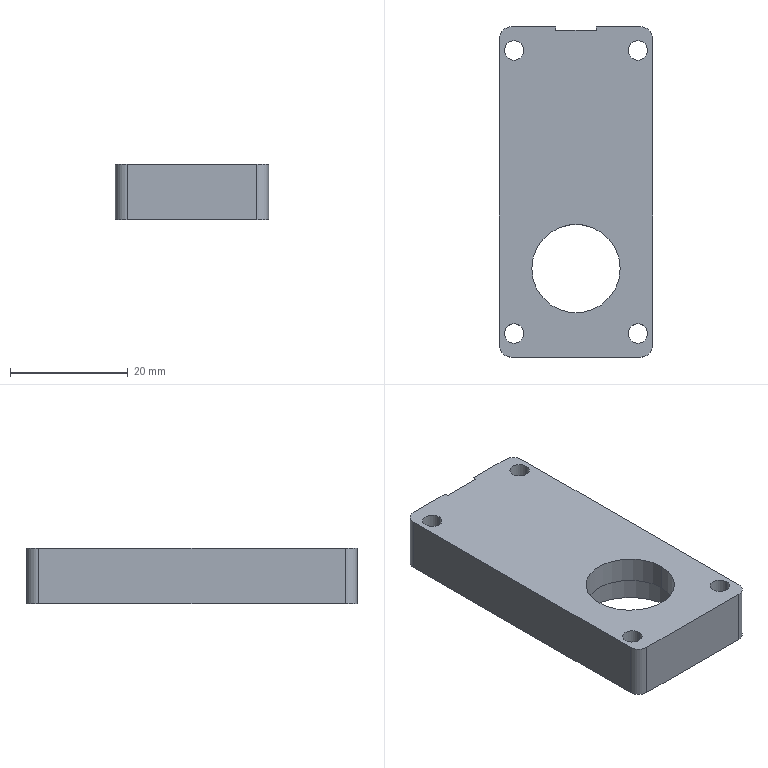Component | SolidWorks | FramePlateSlider.1-1 | 1 solid | 31 faces | box 26 x 56 x 9.4 mm | volume 10956 mm3 | cylinder 20 | plane 9 | cone 2 | commonest cylinder face diameters 3.3 x8 4 x6 19 x2 15 x2 11.6 x2
build123d program:
from build123d import *

# Parameters (mm, degrees)
SKETCH1_2_R           = 7.5
BOSS_EXTRUDE1_DEPTH   = 9.4
M4_TAPPED_HOLE1_D     = 3.3
M4_TAPPED_HOLE1_DEPTH = 10.1
M4_TAPPED_HOLE1_TIP   = 0.9914
M4_TAPPED_HOLE2_D     = 4
M4_TAPPED_HOLE2_DEPTH = 10.1
M4_TAPPED_HOLE2_TIP   = 1.202
SKETCH8_R             = 9.5
CUT_EXTRUDE1_2_DEPTH  = 5
SKETCH1_R             = 5.8
CUT_EXTRUDE1_DEPTH    = 0.6


with BuildPart() as part:
    # Sketch1_2 → Boss-Extrude1 (new body)
    with BuildSketch(Plane.XY):
        with BuildLine():
            Line((-11, 56), (11, 56))
            ThreePointArc((11, 56), (12.414, 55.414), (13, 54))
            Line((13, 54), (13, 2))
            ThreePointArc((13, 2), (12.414, 0.5858), (11, 0))
            Line((11, 0), (-11, 0))
            ThreePointArc((-11, 0), (-12.414, 0.5858), (-13, 2))
            Line((-13, 2), (-13, 54))
            ThreePointArc((-13, 54), (-12.414, 55.414), (-11, 56))
        make_face()
        with Locations((0, 15)):
            Circle(SKETCH1_2_R, mode=Mode.SUBTRACT)
    extrude(amount=BOSS_EXTRUDE1_DEPTH)

    # M4 Tapped Hole1
    with Locations(Plane(origin=(8.389, 4.857, 9.4), x_dir=(1, 0, 0), z_dir=(0, 0, 1))):
        with Locations((-18.889, 47.143), (2.111, 47.143), (-18.889, -0.8568), (2.111, -0.8568)):
            Hole(M4_TAPPED_HOLE1_D / 2, depth=M4_TAPPED_HOLE1_DEPTH)
            with Locations((0, 0, -(M4_TAPPED_HOLE1_DEPTH + M4_TAPPED_HOLE1_TIP / 2))):  # 118° drill point
                Cone(0, M4_TAPPED_HOLE1_D / 2, M4_TAPPED_HOLE1_TIP, mode=Mode.SUBTRACT)

    # M4 Tapped Hole2
    with Locations(Plane(origin=(0, 56, 0), x_dir=(-1, 0, 0), z_dir=(0, 1, 0))):
        with Locations((0, 4.7)):
            Hole(M4_TAPPED_HOLE2_D / 2, depth=M4_TAPPED_HOLE2_DEPTH)
            with Locations((0, 0, -(M4_TAPPED_HOLE2_DEPTH + M4_TAPPED_HOLE2_TIP / 2))):  # 118° drill point
                Cone(0, M4_TAPPED_HOLE2_D / 2, M4_TAPPED_HOLE2_TIP, mode=Mode.SUBTRACT)

    # Sketch8 → Cut-Extrude1_2 (cut)
    with BuildSketch(Plane.XY.offset(9.4)):
        with Locations((0, 15)):
            Circle(SKETCH8_R)
    extrude(amount=-CUT_EXTRUDE1_2_DEPTH, mode=Mode.SUBTRACT)

    # Sketch1 → Cut-Extrude1 (cut, symmetric)
    with BuildSketch(Plane(origin=(0, 56, 0), x_dir=(1, 0, 0), z_dir=(0, 1, 0))):
        with Locations((0, -4.7)):
            Circle(SKETCH1_R)
    extrude(amount=CUT_EXTRUDE1_DEPTH, both=True, mode=Mode.SUBTRACT)


solid = part.part

# Placed as in the assembly
solid = solid.moved(Location((40.5, 151.5, 79.4), (-180, 0, 180)))
STEP:
#1=COLOUR_RGB('',0.7922,0.8196,0.9333);
#2=FILL_AREA_STYLE_COLOUR('',#1);
#3=FILL_AREA_STYLE('',(#2));
#4=SURFACE_STYLE_FILL_AREA(#3);
#5=SURFACE_SIDE_STYLE('',(#4));
#6=SURFACE_STYLE_USAGE(.BOTH.,#5);
#7=PRESENTATION_STYLE_ASSIGNMENT((#6));
#8=CARTESIAN_POINT('',(1.594,7.772,3.02));
#9=VERTEX_POINT('',#8);
#10=CARTESIAN_POINT('',(1.594,7.772,2.862));
#11=VERTEX_POINT('',#10);
#12=CARTESIAN_POINT('',(1.594,7.772,2.941));
#13=DIRECTION('',(-0.,1.,-0.));
#14=DIRECTION('',(0.,0.,-1.));
#15=AXIS2_PLACEMENT_3D('',#12,#13,#14);
#16=CIRCLE('',#15,0.07874);
#17=EDGE_CURVE('',#9,#11,#16,.T.);
#18=ORIENTED_EDGE('',*,*,#17,.F.);
#19=CARTESIAN_POINT('',(1.594,8.146,3.02));
#20=VERTEX_POINT('',#19);
#21=CARTESIAN_POINT('',(1.594,8.169,3.02));
#22=DIRECTION('',(-0.,1.,-0.));
#23=VECTOR('',#22,39.37);
#24=LINE('',#21,#23);
#25=EDGE_CURVE('',#9,#20,#24,.T.);
#26=ORIENTED_EDGE('',*,*,#25,.T.);
#27=CARTESIAN_POINT('',(1.594,8.146,2.862));
#28=VERTEX_POINT('',#27);
#29=CARTESIAN_POINT('',(1.594,8.146,2.941));
#30=DIRECTION('',(0.,-1.,0.));
#31=DIRECTION('',(0.,0.,-1.));
#32=AXIS2_PLACEMENT_3D('',#29,#30,#31);
#33=CIRCLE('',#32,0.07874);
#34=EDGE_CURVE('',#28,#20,#33,.T.);
#35=ORIENTED_EDGE('',*,*,#34,.F.);
#36=CARTESIAN_POINT('',(1.594,8.169,2.862));
#37=DIRECTION('',(-0.,1.,-0.));
#38=VECTOR('',#37,39.37);
#39=LINE('',#36,#38);
#40=EDGE_CURVE('',#11,#28,#39,.T.);
#41=ORIENTED_EDGE('',*,*,#40,.F.);
#42=EDGE_LOOP('',(#18,#26,#35,#41));
#43=FACE_OUTER_BOUND('',#42,.T.);
#44=CARTESIAN_POINT('',(1.594,8.169,2.941));
#45=DIRECTION('',(-0.,1.,-0.));
#46=DIRECTION('',(0.,0.,-1.));
#47=AXIS2_PLACEMENT_3D('',#44,#45,#46);
#48=CYLINDRICAL_SURFACE('',#47,0.07874);
#49=ADVANCED_FACE('',(#43),#48,.F.);
#50=CARTESIAN_POINT('',(1.594,7.724,2.941));
#51=VERTEX_POINT('',#50);
#52=CARTESIAN_POINT('',(1.594,7.772,2.862));
#53=DIRECTION('',(0.,0.515,-0.8572));
#54=VECTOR('',#53,39.37);
#55=LINE('',#52,#54);
#56=EDGE_CURVE('',#51,#11,#55,.T.);
#57=ORIENTED_EDGE('',*,*,#56,.F.);
#58=CARTESIAN_POINT('',(1.594,7.772,3.02));
#59=DIRECTION('',(-0.,0.515,0.8572));
#60=VECTOR('',#59,39.37);
#61=LINE('',#58,#60);
#62=EDGE_CURVE('',#51,#9,#61,.T.);
#63=ORIENTED_EDGE('',*,*,#62,.T.);
#64=ORIENTED_EDGE('',*,*,#17,.T.);
#65=EDGE_LOOP('',(#57,#63,#64));
#66=FACE_OUTER_BOUND('',#65,.T.);
#67=CARTESIAN_POINT('',(1.594,7.772,2.941));
#68=DIRECTION('',(-0.,1.,-0.));
#69=DIRECTION('',(0.,0.,-1.));
#70=AXIS2_PLACEMENT_3D('',#67,#68,#69);
#71=CONICAL_SURFACE('',#70,0.07874,1.03);
#72=ADVANCED_FACE('',(#66),#71,.F.);
#73=CARTESIAN_POINT('',(1.969,6.555,2.953));
#74=VERTEX_POINT('',#73);
#75=CARTESIAN_POINT('',(1.22,6.555,2.953));
#76=VERTEX_POINT('',#75);
#77=CARTESIAN_POINT('',(1.594,6.555,2.953));
#78=DIRECTION('',(0.,-0.,-1.));
#79=DIRECTION('',(-1.,0.,0.));
#80=AXIS2_PLACEMENT_3D('',#77,#78,#79);
#81=CIRCLE('',#80,0.374);
#82=EDGE_CURVE('',#74,#76,#81,.T.);
#83=ORIENTED_EDGE('',*,*,#82,.F.);
#84=CARTESIAN_POINT('',(1.969,6.555,2.756));
#85=VERTEX_POINT('',#84);
#86=CARTESIAN_POINT('',(1.969,6.555,2.953));
#87=DIRECTION('',(0.,-0.,-1.));
#88=VECTOR('',#87,39.37);
#89=LINE('',#86,#88);
#90=EDGE_CURVE('',#74,#85,#89,.T.);
#91=ORIENTED_EDGE('',*,*,#90,.T.);
#92=CARTESIAN_POINT('',(1.22,6.555,2.756));
#93=VERTEX_POINT('',#92);
#94=CARTESIAN_POINT('',(1.594,6.555,2.756));
#95=DIRECTION('',(0.,-0.,-1.));
#96=DIRECTION('',(-1.,0.,0.));
#97=AXIS2_PLACEMENT_3D('',#94,#95,#96);
#98=CIRCLE('',#97,0.374);
#99=EDGE_CURVE('',#85,#93,#98,.T.);
#100=ORIENTED_EDGE('',*,*,#99,.T.);
#101=CARTESIAN_POINT('',(1.22,6.555,2.953));
#102=DIRECTION('',(0.,-0.,-1.));
#103=VECTOR('',#102,39.37);
#104=LINE('',#101,#103);
#105=EDGE_CURVE('',#76,#93,#104,.T.);
#106=ORIENTED_EDGE('',*,*,#105,.F.);
#107=EDGE_LOOP('',(#83,#91,#100,#106));
#108=FACE_OUTER_BOUND('',#107,.T.);
#109=CARTESIAN_POINT('',(1.594,6.555,2.953));
#110=DIRECTION('',(0.,-0.,-1.));
#111=DIRECTION('',(-1.,0.,0.));
#112=AXIS2_PLACEMENT_3D('',#109,#110,#111);
#113=CYLINDRICAL_SURFACE('',#112,0.374);
#114=ADVANCED_FACE('',(#108),#113,.F.);
#115=CARTESIAN_POINT('',(2.073,8.012,3.126));
#116=VERTEX_POINT('',#115);
#117=CARTESIAN_POINT('',(1.943,8.012,3.126));
#118=VERTEX_POINT('',#117);
#119=CARTESIAN_POINT('',(2.008,8.012,3.126));
#120=DIRECTION('',(0.,-0.,-1.));
#121=DIRECTION('',(-1.,0.,0.));
#122=AXIS2_PLACEMENT_3D('',#119,#120,#121);
#123=CIRCLE('',#122,0.06496);
#124=EDGE_CURVE('',#116,#118,#123,.T.);
#125=ORIENTED_EDGE('',*,*,#124,.F.);
#126=CARTESIAN_POINT('',(2.073,8.012,2.756));
#127=VERTEX_POINT('',#126);
#128=CARTESIAN_POINT('',(2.073,8.012,2.756));
#129=DIRECTION('',(0.,-0.,-1.));
#130=VECTOR('',#129,39.37);
#131=LINE('',#128,#130);
#132=EDGE_CURVE('',#116,#127,#131,.T.);
#133=ORIENTED_EDGE('',*,*,#132,.T.);
#134=CARTESIAN_POINT('',(1.943,8.012,2.756));
#135=VERTEX_POINT('',#134);
#136=CARTESIAN_POINT('',(2.008,8.012,2.756));
#137=DIRECTION('',(0.,-0.,-1.));
#138=DIRECTION('',(-1.,0.,0.));
#139=AXIS2_PLACEMENT_3D('',#136,#137,#138);
#140=CIRCLE('',#139,0.06496);
#141=EDGE_CURVE('',#127,#135,#140,.T.);
#142=ORIENTED_EDGE('',*,*,#141,.T.);
#143=CARTESIAN_POINT('',(1.943,8.012,2.756));
#144=DIRECTION('',(0.,-0.,-1.));
#145=VECTOR('',#144,39.37);
#146=LINE('',#143,#145);
#147=EDGE_CURVE('',#118,#135,#146,.T.);
#148=ORIENTED_EDGE('',*,*,#147,.F.);
#149=EDGE_LOOP('',(#125,#133,#142,#148));
#150=FACE_OUTER_BOUND('',#149,.T.);
#151=CARTESIAN_POINT('',(2.008,8.012,2.756));
#152=DIRECTION('',(0.,-0.,-1.));
#153=DIRECTION('',(-1.,0.,0.));
#154=AXIS2_PLACEMENT_3D('',#151,#152,#153);
#155=CYLINDRICAL_SURFACE('',#154,0.06496);
#156=ADVANCED_FACE('',(#150),#155,.F.);
#157=CARTESIAN_POINT('',(1.246,8.012,3.126));
#158=VERTEX_POINT('',#157);
#159=CARTESIAN_POINT('',(1.116,8.012,3.126));
#160=VERTEX_POINT('',#159);
#161=CARTESIAN_POINT('',(1.181,8.012,3.126));
#162=DIRECTION('',(0.,-0.,-1.));
#163=DIRECTION('',(-1.,0.,0.));
#164=AXIS2_PLACEMENT_3D('',#161,#162,#163);
#165=CIRCLE('',#164,0.06496);
#166=EDGE_CURVE('',#158,#160,#165,.T.);
#167=ORIENTED_EDGE('',*,*,#166,.F.);
#168=CARTESIAN_POINT('',(1.246,8.012,2.756));
#169=VERTEX_POINT('',#168);
#170=CARTESIAN_POINT('',(1.246,8.012,2.756));
#171=DIRECTION('',(0.,-0.,-1.));
#172=VECTOR('',#171,39.37);
#173=LINE('',#170,#172);
#174=EDGE_CURVE('',#158,#169,#173,.T.);
#175=ORIENTED_EDGE('',*,*,#174,.T.);
#176=CARTESIAN_POINT('',(1.116,8.012,2.756));
#177=VERTEX_POINT('',#176);
#178=CARTESIAN_POINT('',(1.181,8.012,2.756));
#179=DIRECTION('',(0.,-0.,-1.));
#180=DIRECTION('',(-1.,0.,0.));
#181=AXIS2_PLACEMENT_3D('',#178,#179,#180);
#182=CIRCLE('',#181,0.06496);
#183=EDGE_CURVE('',#169,#177,#182,.T.);
#184=ORIENTED_EDGE('',*,*,#183,.T.);
#185=CARTESIAN_POINT('',(1.116,8.012,2.756));
#186=DIRECTION('',(0.,-0.,-1.));
#187=VECTOR('',#186,39.37);
#188=LINE('',#185,#187);
#189=EDGE_CURVE('',#160,#177,#188,.T.);
#190=ORIENTED_EDGE('',*,*,#189,.F.);
#191=EDGE_LOOP('',(#167,#175,#184,#190));
#192=FACE_OUTER_BOUND('',#191,.T.);
#193=CARTESIAN_POINT('',(1.181,8.012,2.756));
#194=DIRECTION('',(0.,-0.,-1.));
#195=DIRECTION('',(-1.,0.,0.));
#196=AXIS2_PLACEMENT_3D('',#193,#194,#195);
#197=CYLINDRICAL_SURFACE('',#196,0.06496);
#198=ADVANCED_FACE('',(#192),#197,.F.);
#199=CARTESIAN_POINT('',(2.073,6.122,3.126));
#200=VERTEX_POINT('',#199);
#201=CARTESIAN_POINT('',(1.943,6.122,3.126));
#202=VERTEX_POINT('',#201);
#203=CARTESIAN_POINT('',(2.008,6.122,3.126));
#204=DIRECTION('',(0.,-0.,-1.));
#205=DIRECTION('',(-1.,0.,0.));
#206=AXIS2_PLACEMENT_3D('',#203,#204,#205);
#207=CIRCLE('',#206,0.06496);
#208=EDGE_CURVE('',#200,#202,#207,.T.);
#209=ORIENTED_EDGE('',*,*,#208,.F.);
#210=CARTESIAN_POINT('',(2.073,6.122,2.756));
#211=VERTEX_POINT('',#210);
#212=CARTESIAN_POINT('',(2.073,6.122,2.756));
#213=DIRECTION('',(0.,-0.,-1.));
#214=VECTOR('',#213,39.37);
#215=LINE('',#212,#214);
#216=EDGE_CURVE('',#200,#211,#215,.T.);
#217=ORIENTED_EDGE('',*,*,#216,.T.);
#218=CARTESIAN_POINT('',(1.943,6.122,2.756));
#219=VERTEX_POINT('',#218);
#220=CARTESIAN_POINT('',(2.008,6.122,2.756));
#221=DIRECTION('',(0.,-0.,-1.));
#222=DIRECTION('',(-1.,0.,0.));
#223=AXIS2_PLACEMENT_3D('',#220,#221,#222);
#224=CIRCLE('',#223,0.06496);
#225=EDGE_CURVE('',#211,#219,#224,.T.);
#226=ORIENTED_EDGE('',*,*,#225,.T.);
#227=CARTESIAN_POINT('',(1.943,6.122,2.756));
#228=DIRECTION('',(0.,-0.,-1.));
#229=VECTOR('',#228,39.37);
#230=LINE('',#227,#229);
#231=EDGE_CURVE('',#202,#219,#230,.T.);
#232=ORIENTED_EDGE('',*,*,#231,.F.);
#233=EDGE_LOOP('',(#209,#217,#226,#232));
#234=FACE_OUTER_BOUND('',#233,.T.);
#235=CARTESIAN_POINT('',(2.008,6.122,2.756));
#236=DIRECTION('',(0.,-0.,-1.));
#237=DIRECTION('',(-1.,0.,0.));
#238=AXIS2_PLACEMENT_3D('',#235,#236,#237);
#239=CYLINDRICAL_SURFACE('',#238,0.06496);
#240=ADVANCED_FACE('',(#234),#239,.F.);
#241=CARTESIAN_POINT('',(1.246,6.122,3.126));
#242=VERTEX_POINT('',#241);
#243=CARTESIAN_POINT('',(1.116,6.122,3.126));
#244=VERTEX_POINT('',#243);
#245=CARTESIAN_POINT('',(1.181,6.122,3.126));
#246=DIRECTION('',(0.,-0.,-1.));
#247=DIRECTION('',(-1.,0.,0.));
#248=AXIS2_PLACEMENT_3D('',#245,#246,#247);
#249=CIRCLE('',#248,0.06496);
#250=EDGE_CURVE('',#242,#244,#249,.T.);
#251=ORIENTED_EDGE('',*,*,#250,.F.);
#252=CARTESIAN_POINT('',(1.246,6.122,2.756));
#253=VERTEX_POINT('',#252);
#254=CARTESIAN_POINT('',(1.246,6.122,2.756));
#255=DIRECTION('',(0.,-0.,-1.));
#256=VECTOR('',#255,39.37);
#257=LINE('',#254,#256);
#258=EDGE_CURVE('',#242,#253,#257,.T.);
#259=ORIENTED_EDGE('',*,*,#258,.T.);
#260=CARTESIAN_POINT('',(1.116,6.122,2.756));
#261=VERTEX_POINT('',#260);
#262=CARTESIAN_POINT('',(1.181,6.122,2.756));
#263=DIRECTION('',(0.,-0.,-1.));
#264=DIRECTION('',(-1.,0.,0.));
#265=AXIS2_PLACEMENT_3D('',#262,#263,#264);
#266=CIRCLE('',#265,0.06496);
#267=EDGE_CURVE('',#253,#261,#266,.T.);
#268=ORIENTED_EDGE('',*,*,#267,.T.);
#269=CARTESIAN_POINT('',(1.116,6.122,2.756));
#270=DIRECTION('',(0.,-0.,-1.));
#271=VECTOR('',#270,39.37);
#272=LINE('',#269,#271);
#273=EDGE_CURVE('',#244,#261,#272,.T.);
#274=ORIENTED_EDGE('',*,*,#273,.F.);
#275=EDGE_LOOP('',(#251,#259,#268,#274));
#276=FACE_OUTER_BOUND('',#275,.T.);
#277=CARTESIAN_POINT('',(1.181,6.122,2.756));
#278=DIRECTION('',(0.,-0.,-1.));
#279=DIRECTION('',(-1.,0.,0.));
#280=AXIS2_PLACEMENT_3D('',#277,#278,#279);
#281=CYLINDRICAL_SURFACE('',#280,0.06496);
#282=ADVANCED_FACE('',(#276),#281,.F.);
#283=CARTESIAN_POINT('',(1.89,6.555,2.953));
#284=VERTEX_POINT('',#283);
#285=CARTESIAN_POINT('',(1.299,6.555,2.953));
#286=VERTEX_POINT('',#285);
#287=CARTESIAN_POINT('',(1.594,6.555,2.953));
#288=DIRECTION('',(0.,-0.,-1.));
#289=DIRECTION('',(-1.,0.,0.));
#290=AXIS2_PLACEMENT_3D('',#287,#288,#289);
#291=CIRCLE('',#290,0.2953);
#292=EDGE_CURVE('',#284,#286,#291,.T.);
#293=ORIENTED_EDGE('',*,*,#292,.T.);
#294=CARTESIAN_POINT('',(1.299,6.555,3.126));
#295=VERTEX_POINT('',#294);
#296=CARTESIAN_POINT('',(1.299,6.555,2.756));
#297=DIRECTION('',(-0.,0.,1.));
#298=VECTOR('',#297,39.37);
#299=LINE('',#296,#298);
#300=EDGE_CURVE('',#286,#295,#299,.T.);
#301=ORIENTED_EDGE('',*,*,#300,.T.);
#302=CARTESIAN_POINT('',(1.89,6.555,3.126));
#303=VERTEX_POINT('',#302);
#304=CARTESIAN_POINT('',(1.594,6.555,3.126));
#305=DIRECTION('',(0.,-0.,-1.));
#306=DIRECTION('',(-1.,0.,0.));
#307=AXIS2_PLACEMENT_3D('',#304,#305,#306);
#308=CIRCLE('',#307,0.2953);
#309=EDGE_CURVE('',#303,#295,#308,.T.);
#310=ORIENTED_EDGE('',*,*,#309,.F.);
#311=CARTESIAN_POINT('',(1.89,6.555,2.756));
#312=DIRECTION('',(-0.,0.,1.));
#313=VECTOR('',#312,39.37);
#314=LINE('',#311,#313);
#315=EDGE_CURVE('',#284,#303,#314,.T.);
#316=ORIENTED_EDGE('',*,*,#315,.F.);
#317=EDGE_LOOP('',(#293,#301,#310,#316));
#318=FACE_OUTER_BOUND('',#317,.T.);
#319=CARTESIAN_POINT('',(1.594,6.555,2.756));
#320=DIRECTION('',(-0.,0.,1.));
#321=DIRECTION('',(1.,0.,0.));
#322=AXIS2_PLACEMENT_3D('',#319,#320,#321);
#323=CYLINDRICAL_SURFACE('',#322,0.2953);
#324=ADVANCED_FACE('',(#318),#323,.F.);
#325=CARTESIAN_POINT('',(1.161,8.169,3.126));
#326=VERTEX_POINT('',#325);
#327=CARTESIAN_POINT('',(1.461,8.169,3.126));
#328=VERTEX_POINT('',#327);
#329=CARTESIAN_POINT('',(2.028,8.169,3.126));
#330=DIRECTION('',(1.,-0.,0.));
#331=VECTOR('',#330,39.37);
#332=LINE('',#329,#331);
#333=EDGE_CURVE('',#326,#328,#332,.T.);
#334=ORIENTED_EDGE('',*,*,#333,.T.);
#335=CARTESIAN_POINT('',(1.461,8.169,2.756));
#336=VERTEX_POINT('',#335);
#337=CARTESIAN_POINT('',(1.594,8.169,2.941));
#338=DIRECTION('',(0.,-1.,0.));
#339=DIRECTION('',(0.,0.,1.));
#340=AXIS2_PLACEMENT_3D('',#337,#338,#339);
#341=CIRCLE('',#340,0.2283);
#342=EDGE_CURVE('',#328,#336,#341,.T.);
#343=ORIENTED_EDGE('',*,*,#342,.T.);
#344=CARTESIAN_POINT('',(1.161,8.169,2.756));
#345=VERTEX_POINT('',#344);
#346=CARTESIAN_POINT('',(2.028,8.169,2.756));
#347=DIRECTION('',(1.,-0.,0.));
#348=VECTOR('',#347,39.37);
#349=LINE('',#346,#348);
#350=EDGE_CURVE('',#345,#336,#349,.T.);
#351=ORIENTED_EDGE('',*,*,#350,.F.);
#352=CARTESIAN_POINT('',(1.161,8.169,2.756));
#353=DIRECTION('',(-0.,0.,1.));
#354=VECTOR('',#353,39.37);
#355=LINE('',#352,#354);
#356=EDGE_CURVE('',#345,#326,#355,.T.);
#357=ORIENTED_EDGE('',*,*,#356,.T.);
#358=EDGE_LOOP('',(#334,#343,#351,#357));
#359=FACE_OUTER_BOUND('',#358,.T.);
#360=CARTESIAN_POINT('',(2.028,8.169,2.756));
#361=DIRECTION('',(0.,-1.,0.));
#362=DIRECTION('',(-0.,0.,1.));
#363=AXIS2_PLACEMENT_3D('',#360,#361,#362);
#364=PLANE('',#363);
#365=ADVANCED_FACE('',(#359),#364,.F.);
#366=ORIENTED_EDGE('',*,*,#300,.F.);
#367=CARTESIAN_POINT('',(1.594,6.555,2.953));
#368=DIRECTION('',(0.,-0.,-1.));
#369=DIRECTION('',(-1.,0.,0.));
#370=AXIS2_PLACEMENT_3D('',#367,#368,#369);
#371=CIRCLE('',#370,0.2953);
#372=EDGE_CURVE('',#286,#284,#371,.T.);
#373=ORIENTED_EDGE('',*,*,#372,.T.);
#374=ORIENTED_EDGE('',*,*,#315,.T.);
#375=CARTESIAN_POINT('',(1.594,6.555,3.126));
#376=DIRECTION('',(0.,-0.,-1.));
#377=DIRECTION('',(-1.,0.,0.));
#378=AXIS2_PLACEMENT_3D('',#375,#376,#377);
#379=CIRCLE('',#378,0.2953);
#380=EDGE_CURVE('',#295,#303,#379,.T.);
#381=ORIENTED_EDGE('',*,*,#380,.F.);
#382=EDGE_LOOP('',(#366,#373,#374,#381));
#383=FACE_OUTER_BOUND('',#382,.T.);
#384=CARTESIAN_POINT('',(1.594,6.555,2.756));
#385=DIRECTION('',(-0.,0.,1.));
#386=DIRECTION('',(1.,0.,0.));
#387=AXIS2_PLACEMENT_3D('',#384,#385,#386);
#388=CYLINDRICAL_SURFACE('',#387,0.2953);
#389=ADVANCED_FACE('',(#383),#388,.F.);
#390=CARTESIAN_POINT('',(1.461,8.146,2.756));
#391=VERTEX_POINT('',#390);
#392=CARTESIAN_POINT('',(1.461,8.146,2.756));
#393=DIRECTION('',(-0.,1.,-0.));
#394=VECTOR('',#393,39.37);
#395=LINE('',#392,#394);
#396=EDGE_CURVE('',#391,#336,#395,.T.);
#397=ORIENTED_EDGE('',*,*,#396,.F.);
#398=CARTESIAN_POINT('',(1.728,8.146,2.756));
#399=VERTEX_POINT('',#398);
#400=CARTESIAN_POINT('',(1.161,8.146,2.756));
#401=DIRECTION('',(1.,-0.,0.));
#402=VECTOR('',#401,39.37);
#403=LINE('',#400,#402);
#404=EDGE_CURVE('',#391,#399,#403,.T.);
#405=ORIENTED_EDGE('',*,*,#404,.T.);
#406=CARTESIAN_POINT('',(1.728,8.169,2.756));
#407=VERTEX_POINT('',#406);
#408=CARTESIAN_POINT('',(1.728,8.146,2.756));
#409=DIRECTION('',(0.,-1.,0.));
#410=VECTOR('',#409,39.37);
#411=LINE('',#408,#410);
#412=EDGE_CURVE('',#407,#399,#411,.T.);
#413=ORIENTED_EDGE('',*,*,#412,.F.);
#414=CARTESIAN_POINT('',(2.028,8.169,2.756));
#415=VERTEX_POINT('',#414);
#416=CARTESIAN_POINT('',(2.028,8.169,2.756));
#417=DIRECTION('',(1.,-0.,0.));
#418=VECTOR('',#417,39.37);
#419=LINE('',#416,#418);
#420=EDGE_CURVE('',#407,#415,#419,.T.);
#421=ORIENTED_EDGE('',*,*,#420,.T.);
#422=CARTESIAN_POINT('',(2.106,8.091,2.756));
#423=VERTEX_POINT('',#422);
#424=CARTESIAN_POINT('',(2.028,8.091,2.756));
#425=DIRECTION('',(0.,-0.,-1.));
#426=DIRECTION('',(-1.,0.,0.));
#427=AXIS2_PLACEMENT_3D('',#424,#425,#426);
#428=CIRCLE('',#427,0.07874);
#429=EDGE_CURVE('',#415,#423,#428,.T.);
#430=ORIENTED_EDGE('',*,*,#429,.T.);
#431=CARTESIAN_POINT('',(2.106,6.043,2.756));
#432=VERTEX_POINT('',#431);
#433=CARTESIAN_POINT('',(2.106,8.091,2.756));
#434=DIRECTION('',(-0.,-1.,0.));
#435=VECTOR('',#434,39.37);
#436=LINE('',#433,#435);
#437=EDGE_CURVE('',#423,#432,#436,.T.);
#438=ORIENTED_EDGE('',*,*,#437,.T.);
#439=CARTESIAN_POINT('',(2.028,5.965,2.756));
#440=VERTEX_POINT('',#439);
#441=CARTESIAN_POINT('',(2.028,6.043,2.756));
#442=DIRECTION('',(0.,-0.,-1.));
#443=DIRECTION('',(1.,0.,0.));
#444=AXIS2_PLACEMENT_3D('',#441,#442,#443);
#445=CIRCLE('',#444,0.07874);
#446=EDGE_CURVE('',#432,#440,#445,.T.);
#447=ORIENTED_EDGE('',*,*,#446,.T.);
#448=CARTESIAN_POINT('',(1.161,5.965,2.756));
#449=VERTEX_POINT('',#448);
#450=CARTESIAN_POINT('',(2.028,5.965,2.756));
#451=DIRECTION('',(-1.,0.,-0.));
#452=VECTOR('',#451,39.37);
#453=LINE('',#450,#452);
#454=EDGE_CURVE('',#440,#449,#453,.T.);
#455=ORIENTED_EDGE('',*,*,#454,.T.);
#456=CARTESIAN_POINT('',(1.083,6.043,2.756));
#457=VERTEX_POINT('',#456);
#458=CARTESIAN_POINT('',(1.161,6.043,2.756));
#459=DIRECTION('',(0.,-0.,-1.));
#460=DIRECTION('',(-1.,0.,0.));
#461=AXIS2_PLACEMENT_3D('',#458,#459,#460);
#462=CIRCLE('',#461,0.07874);
#463=EDGE_CURVE('',#449,#457,#462,.T.);
#464=ORIENTED_EDGE('',*,*,#463,.T.);
#465=CARTESIAN_POINT('',(1.083,8.091,2.756));
#466=VERTEX_POINT('',#465);
#467=CARTESIAN_POINT('',(1.083,8.091,2.756));
#468=DIRECTION('',(0.,1.,-0.));
#469=VECTOR('',#468,39.37);
#470=LINE('',#467,#469);
#471=EDGE_CURVE('',#457,#466,#470,.T.);
#472=ORIENTED_EDGE('',*,*,#471,.T.);
#473=CARTESIAN_POINT('',(1.161,8.091,2.756));
#474=DIRECTION('',(0.,-0.,-1.));
#475=DIRECTION('',(-1.,0.,0.));
#476=AXIS2_PLACEMENT_3D('',#473,#474,#475);
#477=CIRCLE('',#476,0.07874);
#478=EDGE_CURVE('',#466,#345,#477,.T.);
#479=ORIENTED_EDGE('',*,*,#478,.T.);
#480=ORIENTED_EDGE('',*,*,#350,.T.);
#481=EDGE_LOOP('',(#397,#405,#413,#421,#430,#438,#447,#455,#464,#472,#479,#480));
#482=FACE_OUTER_BOUND('',#481,.T.);
#483=CARTESIAN_POINT('',(1.594,6.555,2.756));
#484=DIRECTION('',(0.,-0.,-1.));
#485=DIRECTION('',(-1.,0.,0.));
#486=AXIS2_PLACEMENT_3D('',#483,#484,#485);
#487=CIRCLE('',#486,0.374);
#488=EDGE_CURVE('',#93,#85,#487,.T.);
#489=ORIENTED_EDGE('',*,*,#488,.F.);
#490=ORIENTED_EDGE('',*,*,#99,.F.);
#491=EDGE_LOOP('',(#489,#490));
#492=FACE_BOUND('',#491,.T.);
#493=CARTESIAN_POINT('',(2.008,8.012,2.756));
#494=DIRECTION('',(0.,-0.,-1.));
#495=DIRECTION('',(-1.,0.,0.));
#496=AXIS2_PLACEMENT_3D('',#493,#494,#495);
#497=CIRCLE('',#496,0.06496);
#498=EDGE_CURVE('',#135,#127,#497,.T.);
#499=ORIENTED_EDGE('',*,*,#498,.F.);
#500=ORIENTED_EDGE('',*,*,#141,.F.);
#501=EDGE_LOOP('',(#499,#500));
#502=FACE_BOUND('',#501,.T.);
#503=CARTESIAN_POINT('',(1.181,8.012,2.756));
#504=DIRECTION('',(0.,-0.,-1.));
#505=DIRECTION('',(-1.,0.,0.));
#506=AXIS2_PLACEMENT_3D('',#503,#504,#505);
#507=CIRCLE('',#506,0.06496);
#508=EDGE_CURVE('',#177,#169,#507,.T.);
#509=ORIENTED_EDGE('',*,*,#508,.F.);
#510=ORIENTED_EDGE('',*,*,#183,.F.);
#511=EDGE_LOOP('',(#509,#510));
#512=FACE_BOUND('',#511,.T.);
#513=CARTESIAN_POINT('',(2.008,6.122,2.756));
#514=DIRECTION('',(0.,-0.,-1.));
#515=DIRECTION('',(-1.,0.,0.));
#516=AXIS2_PLACEMENT_3D('',#513,#514,#515);
#517=CIRCLE('',#516,0.06496);
#518=EDGE_CURVE('',#219,#211,#517,.T.);
#519=ORIENTED_EDGE('',*,*,#518,.F.);
#520=ORIENTED_EDGE('',*,*,#225,.F.);
#521=EDGE_LOOP('',(#519,#520));
#522=FACE_BOUND('',#521,.T.);
#523=CARTESIAN_POINT('',(1.181,6.122,2.756));
#524=DIRECTION('',(0.,-0.,-1.));
#525=DIRECTION('',(-1.,0.,0.));
#526=AXIS2_PLACEMENT_3D('',#523,#524,#525);
#527=CIRCLE('',#526,0.06496);
#528=EDGE_CURVE('',#261,#253,#527,.T.);
#529=ORIENTED_EDGE('',*,*,#528,.F.);
#530=ORIENTED_EDGE('',*,*,#267,.F.);
#531=EDGE_LOOP('',(#529,#530));
#532=FACE_BOUND('',#531,.T.);
#533=CARTESIAN_POINT('',(1.161,6.043,2.756));
#534=DIRECTION('',(0.,-0.,-1.));
#535=DIRECTION('',(-1.,0.,-0.));
#536=AXIS2_PLACEMENT_3D('',#533,#534,#535);
#537=PLANE('',#536);
#538=ADVANCED_FACE('',(#482,#492,#502,#512,#522,#532),#537,.T.);
#539=CARTESIAN_POINT('',(2.008,8.012,3.126));
#540=DIRECTION('',(0.,-0.,-1.));
#541=DIRECTION('',(-1.,0.,0.));
#542=AXIS2_PLACEMENT_3D('',#539,#540,#541);
#543=CIRCLE('',#542,0.06496);
#544=EDGE_CURVE('',#118,#116,#543,.T.);
#545=ORIENTED_EDGE('',*,*,#544,.T.);
#546=ORIENTED_EDGE('',*,*,#124,.T.);
#547=EDGE_LOOP('',(#545,#546));
#548=FACE_BOUND('',#547,.T.);
#549=CARTESIAN_POINT('',(1.181,8.012,3.126));
#550=DIRECTION('',(0.,-0.,-1.));
#551=DIRECTION('',(-1.,0.,0.));
#552=AXIS2_PLACEMENT_3D('',#549,#550,#551);
#553=CIRCLE('',#552,0.06496);
#554=EDGE_CURVE('',#160,#158,#553,.T.);
#555=ORIENTED_EDGE('',*,*,#554,.T.);
#556=ORIENTED_EDGE('',*,*,#166,.T.);
#557=EDGE_LOOP('',(#555,#556));
#558=FACE_BOUND('',#557,.T.);
#559=CARTESIAN_POINT('',(2.008,6.122,3.126));
#560=DIRECTION('',(0.,-0.,-1.));
#561=DIRECTION('',(-1.,0.,0.));
#562=AXIS2_PLACEMENT_3D('',#559,#560,#561);
#563=CIRCLE('',#562,0.06496);
#564=EDGE_CURVE('',#202,#200,#563,.T.);
#565=ORIENTED_EDGE('',*,*,#564,.T.);
#566=ORIENTED_EDGE('',*,*,#208,.T.);
#567=EDGE_LOOP('',(#565,#566));
#568=FACE_BOUND('',#567,.T.);
#569=CARTESIAN_POINT('',(1.181,6.122,3.126));
#570=DIRECTION('',(0.,-0.,-1.));
#571=DIRECTION('',(-1.,0.,0.));
#572=AXIS2_PLACEMENT_3D('',#569,#570,#571);
#573=CIRCLE('',#572,0.06496);
#574=EDGE_CURVE('',#244,#242,#573,.T.);
#575=ORIENTED_EDGE('',*,*,#574,.T.);
#576=ORIENTED_EDGE('',*,*,#250,.T.);
#577=EDGE_LOOP('',(#575,#576));
#578=FACE_BOUND('',#577,.T.);
#579=CARTESIAN_POINT('',(1.461,8.146,3.126));
#580=VERTEX_POINT('',#579);
#581=CARTESIAN_POINT('',(1.728,8.146,3.126));
#582=VERTEX_POINT('',#581);
#583=CARTESIAN_POINT('',(1.161,8.146,3.126));
#584=DIRECTION('',(1.,-0.,0.));
#585=VECTOR('',#584,39.37);
#586=LINE('',#583,#585);
#587=EDGE_CURVE('',#580,#582,#586,.T.);
#588=ORIENTED_EDGE('',*,*,#587,.F.);
#589=CARTESIAN_POINT('',(1.461,8.146,3.126));
#590=DIRECTION('',(-0.,1.,-0.));
#591=VECTOR('',#590,39.37);
#592=LINE('',#589,#591);
#593=EDGE_CURVE('',#580,#328,#592,.T.);
#594=ORIENTED_EDGE('',*,*,#593,.T.);
#595=ORIENTED_EDGE('',*,*,#333,.F.);
#596=CARTESIAN_POINT('',(1.083,8.091,3.126));
#597=VERTEX_POINT('',#596);
#598=CARTESIAN_POINT('',(1.161,8.091,3.126));
#599=DIRECTION('',(0.,-0.,-1.));
#600=DIRECTION('',(-1.,0.,0.));
#601=AXIS2_PLACEMENT_3D('',#598,#599,#600);
#602=CIRCLE('',#601,0.07874);
#603=EDGE_CURVE('',#597,#326,#602,.T.);
#604=ORIENTED_EDGE('',*,*,#603,.F.);
#605=CARTESIAN_POINT('',(1.083,6.043,3.126));
#606=VERTEX_POINT('',#605);
#607=CARTESIAN_POINT('',(1.083,8.091,3.126));
#608=DIRECTION('',(0.,1.,-0.));
#609=VECTOR('',#608,39.37);
#610=LINE('',#607,#609);
#611=EDGE_CURVE('',#606,#597,#610,.T.);
#612=ORIENTED_EDGE('',*,*,#611,.F.);
#613=CARTESIAN_POINT('',(1.161,5.965,3.126));
#614=VERTEX_POINT('',#613);
#615=CARTESIAN_POINT('',(1.161,6.043,3.126));
#616=DIRECTION('',(0.,-0.,-1.));
#617=DIRECTION('',(-1.,0.,0.));
#618=AXIS2_PLACEMENT_3D('',#615,#616,#617);
#619=CIRCLE('',#618,0.07874);
#620=EDGE_CURVE('',#614,#606,#619,.T.);
#621=ORIENTED_EDGE('',*,*,#620,.F.);
#622=CARTESIAN_POINT('',(2.028,5.965,3.126));
#623=VERTEX_POINT('',#622);
#624=CARTESIAN_POINT('',(2.028,5.965,3.126));
#625=DIRECTION('',(-1.,0.,-0.));
#626=VECTOR('',#625,39.37);
#627=LINE('',#624,#626);
#628=EDGE_CURVE('',#623,#614,#627,.T.);
#629=ORIENTED_EDGE('',*,*,#628,.F.);
#630=CARTESIAN_POINT('',(2.106,6.043,3.126));
#631=VERTEX_POINT('',#630);
#632=CARTESIAN_POINT('',(2.028,6.043,3.126));
#633=DIRECTION('',(0.,-0.,-1.));
#634=DIRECTION('',(1.,0.,0.));
#635=AXIS2_PLACEMENT_3D('',#632,#633,#634);
#636=CIRCLE('',#635,0.07874);
#637=EDGE_CURVE('',#631,#623,#636,.T.);
#638=ORIENTED_EDGE('',*,*,#637,.F.);
#639=CARTESIAN_POINT('',(2.106,8.091,3.126));
#640=VERTEX_POINT('',#639);
#641=CARTESIAN_POINT('',(2.106,8.091,3.126));
#642=DIRECTION('',(-0.,-1.,0.));
#643=VECTOR('',#642,39.37);
#644=LINE('',#641,#643);
#645=EDGE_CURVE('',#640,#631,#644,.T.);
#646=ORIENTED_EDGE('',*,*,#645,.F.);
#647=CARTESIAN_POINT('',(2.028,8.169,3.126));
#648=VERTEX_POINT('',#647);
#649=CARTESIAN_POINT('',(2.028,8.091,3.126));
#650=DIRECTION('',(0.,-0.,-1.));
#651=DIRECTION('',(-1.,0.,0.));
#652=AXIS2_PLACEMENT_3D('',#649,#650,#651);
#653=CIRCLE('',#652,0.07874);
#654=EDGE_CURVE('',#648,#640,#653,.T.);
#655=ORIENTED_EDGE('',*,*,#654,.F.);
#656=CARTESIAN_POINT('',(1.728,8.169,3.126));
#657=VERTEX_POINT('',#656);
#658=CARTESIAN_POINT('',(2.028,8.169,3.126));
#659=DIRECTION('',(1.,-0.,0.));
#660=VECTOR('',#659,39.37);
#661=LINE('',#658,#660);
#662=EDGE_CURVE('',#657,#648,#661,.T.);
#663=ORIENTED_EDGE('',*,*,#662,.F.);
#664=CARTESIAN_POINT('',(1.728,8.146,3.126));
#665=DIRECTION('',(0.,-1.,0.));
#666=VECTOR('',#665,39.37);
#667=LINE('',#664,#666);
#668=EDGE_CURVE('',#657,#582,#667,.T.);
#669=ORIENTED_EDGE('',*,*,#668,.T.);
#670=EDGE_LOOP('',(#588,#594,#595,#604,#612,#621,#629,#638,#646,#655,#663,#669));
#671=FACE_OUTER_BOUND('',#670,.T.);
#672=ORIENTED_EDGE('',*,*,#309,.T.);
#673=ORIENTED_EDGE('',*,*,#380,.T.);
#674=EDGE_LOOP('',(#672,#673));
#675=FACE_BOUND('',#674,.T.);
#676=CARTESIAN_POINT('',(1.161,6.043,3.126));
#677=DIRECTION('',(0.,-0.,-1.));
#678=DIRECTION('',(-1.,0.,-0.));
#679=AXIS2_PLACEMENT_3D('',#676,#677,#678);
#680=PLANE('',#679);
#681=ADVANCED_FACE('',(#548,#558,#568,#578,#671,#675),#680,.F.);
#682=ORIENTED_EDGE('',*,*,#620,.T.);
#683=CARTESIAN_POINT('',(1.083,6.043,2.756));
#684=DIRECTION('',(-0.,0.,1.));
#685=VECTOR('',#684,39.37);
#686=LINE('',#683,#685);
#687=EDGE_CURVE('',#457,#606,#686,.T.);
#688=ORIENTED_EDGE('',*,*,#687,.F.);
#689=ORIENTED_EDGE('',*,*,#463,.F.);
#690=CARTESIAN_POINT('',(1.161,5.965,2.756));
#691=DIRECTION('',(-0.,0.,1.));
#692=VECTOR('',#691,39.37);
#693=LINE('',#690,#692);
#694=EDGE_CURVE('',#449,#614,#693,.T.);
#695=ORIENTED_EDGE('',*,*,#694,.T.);
#696=EDGE_LOOP('',(#682,#688,#689,#695));
#697=FACE_OUTER_BOUND('',#696,.T.);
#698=CARTESIAN_POINT('',(1.161,6.043,2.756));
#699=DIRECTION('',(-0.,0.,1.));
#700=DIRECTION('',(1.,0.,0.));
#701=AXIS2_PLACEMENT_3D('',#698,#699,#700);
#702=CYLINDRICAL_SURFACE('',#701,0.07874);
#703=ADVANCED_FACE('',(#697),#702,.T.);
#704=ORIENTED_EDGE('',*,*,#611,.T.);
#705=CARTESIAN_POINT('',(1.083,8.091,2.756));
#706=DIRECTION('',(-0.,0.,1.));
#707=VECTOR('',#706,39.37);
#708=LINE('',#705,#707);
#709=EDGE_CURVE('',#466,#597,#708,.T.);
#710=ORIENTED_EDGE('',*,*,#709,.F.);
#711=ORIENTED_EDGE('',*,*,#471,.F.);
#712=ORIENTED_EDGE('',*,*,#687,.T.);
#713=EDGE_LOOP('',(#704,#710,#711,#712));
#714=FACE_OUTER_BOUND('',#713,.T.);
#715=CARTESIAN_POINT('',(1.083,8.091,2.756));
#716=DIRECTION('',(1.,-0.,0.));
#717=DIRECTION('',(-0.,-1.,0.));
#718=AXIS2_PLACEMENT_3D('',#715,#716,#717);
#719=PLANE('',#718);
#720=ADVANCED_FACE('',(#714),#719,.F.);
#721=ORIENTED_EDGE('',*,*,#603,.T.);
#722=ORIENTED_EDGE('',*,*,#356,.F.);
#723=ORIENTED_EDGE('',*,*,#478,.F.);
#724=ORIENTED_EDGE('',*,*,#709,.T.);
#725=EDGE_LOOP('',(#721,#722,#723,#724));
#726=FACE_OUTER_BOUND('',#725,.T.);
#727=CARTESIAN_POINT('',(1.161,8.091,2.756));
#728=DIRECTION('',(-0.,0.,1.));
#729=DIRECTION('',(1.,0.,0.));
#730=AXIS2_PLACEMENT_3D('',#727,#728,#729);
#731=CYLINDRICAL_SURFACE('',#730,0.07874);
#732=ADVANCED_FACE('',(#726),#731,.T.);
#733=ORIENTED_EDGE('',*,*,#420,.F.);
#734=CARTESIAN_POINT('',(1.594,8.169,2.941));
#735=DIRECTION('',(0.,-1.,0.));
#736=DIRECTION('',(0.,0.,1.));
#737=AXIS2_PLACEMENT_3D('',#734,#735,#736);
#738=CIRCLE('',#737,0.2283);
#739=EDGE_CURVE('',#407,#657,#738,.T.);
#740=ORIENTED_EDGE('',*,*,#739,.T.);
#741=ORIENTED_EDGE('',*,*,#662,.T.);
#742=CARTESIAN_POINT('',(2.028,8.169,2.756));
#743=DIRECTION('',(-0.,0.,1.));
#744=VECTOR('',#743,39.37);
#745=LINE('',#742,#744);
#746=EDGE_CURVE('',#415,#648,#745,.T.);
#747=ORIENTED_EDGE('',*,*,#746,.F.);
#748=EDGE_LOOP('',(#733,#740,#741,#747));
#749=FACE_OUTER_BOUND('',#748,.T.);
#750=CARTESIAN_POINT('',(2.028,8.169,2.756));
#751=DIRECTION('',(0.,-1.,0.));
#752=DIRECTION('',(-0.,0.,1.));
#753=AXIS2_PLACEMENT_3D('',#750,#751,#752);
#754=PLANE('',#753);
#755=ADVANCED_FACE('',(#749),#754,.F.);
#756=ORIENTED_EDGE('',*,*,#654,.T.);
#757=CARTESIAN_POINT('',(2.106,8.091,2.756));
#758=DIRECTION('',(-0.,0.,1.));
#759=VECTOR('',#758,39.37);
#760=LINE('',#757,#759);
#761=EDGE_CURVE('',#423,#640,#760,.T.);
#762=ORIENTED_EDGE('',*,*,#761,.F.);
#763=ORIENTED_EDGE('',*,*,#429,.F.);
#764=ORIENTED_EDGE('',*,*,#746,.T.);
#765=EDGE_LOOP('',(#756,#762,#763,#764));
#766=FACE_OUTER_BOUND('',#765,.T.);
#767=CARTESIAN_POINT('',(2.028,8.091,2.756));
#768=DIRECTION('',(-0.,0.,1.));
#769=DIRECTION('',(1.,0.,0.));
#770=AXIS2_PLACEMENT_3D('',#767,#768,#769);
#771=CYLINDRICAL_SURFACE('',#770,0.07874);
#772=ADVANCED_FACE('',(#766),#771,.T.);
#773=ORIENTED_EDGE('',*,*,#645,.T.);
#774=CARTESIAN_POINT('',(2.106,6.043,2.756));
#775=DIRECTION('',(-0.,0.,1.));
#776=VECTOR('',#775,39.37);
#777=LINE('',#774,#776);
#778=EDGE_CURVE('',#432,#631,#777,.T.);
#779=ORIENTED_EDGE('',*,*,#778,.F.);
#780=ORIENTED_EDGE('',*,*,#437,.F.);
#781=ORIENTED_EDGE('',*,*,#761,.T.);
#782=EDGE_LOOP('',(#773,#779,#780,#781));
#783=FACE_OUTER_BOUND('',#782,.T.);
#784=CARTESIAN_POINT('',(2.106,8.091,2.756));
#785=DIRECTION('',(-1.,0.,-0.));
#786=DIRECTION('',(0.,1.,-0.));
#787=AXIS2_PLACEMENT_3D('',#784,#785,#786);
#788=PLANE('',#787);
#789=ADVANCED_FACE('',(#783),#788,.F.);
#790=ORIENTED_EDGE('',*,*,#637,.T.);
#791=CARTESIAN_POINT('',(2.028,5.965,2.756));
#792=DIRECTION('',(-0.,0.,1.));
#793=VECTOR('',#792,39.37);
#794=LINE('',#791,#793);
#795=EDGE_CURVE('',#440,#623,#794,.T.);
#796=ORIENTED_EDGE('',*,*,#795,.F.);
#797=ORIENTED_EDGE('',*,*,#446,.F.);
#798=ORIENTED_EDGE('',*,*,#778,.T.);
#799=EDGE_LOOP('',(#790,#796,#797,#798));
#800=FACE_OUTER_BOUND('',#799,.T.);
#801=CARTESIAN_POINT('',(2.028,6.043,2.756));
#802=DIRECTION('',(-0.,0.,1.));
#803=DIRECTION('',(1.,0.,0.));
#804=AXIS2_PLACEMENT_3D('',#801,#802,#803);
#805=CYLINDRICAL_SURFACE('',#804,0.07874);
#806=ADVANCED_FACE('',(#800),#805,.T.);
#807=ORIENTED_EDGE('',*,*,#628,.T.);
#808=ORIENTED_EDGE('',*,*,#694,.F.);
#809=ORIENTED_EDGE('',*,*,#454,.F.);
#810=ORIENTED_EDGE('',*,*,#795,.T.);
#811=EDGE_LOOP('',(#807,#808,#809,#810));
#812=FACE_OUTER_BOUND('',#811,.T.);
#813=CARTESIAN_POINT('',(2.028,5.965,2.756));
#814=DIRECTION('',(-0.,1.,-0.));
#815=DIRECTION('',(0.,-0.,-1.));
#816=AXIS2_PLACEMENT_3D('',#813,#814,#815);
#817=PLANE('',#816);
#818=ADVANCED_FACE('',(#812),#817,.F.);
#819=ORIENTED_EDGE('',*,*,#258,.F.);
#820=ORIENTED_EDGE('',*,*,#574,.F.);
#821=ORIENTED_EDGE('',*,*,#273,.T.);
#822=ORIENTED_EDGE('',*,*,#528,.T.);
#823=EDGE_LOOP('',(#819,#820,#821,#822));
#824=FACE_OUTER_BOUND('',#823,.T.);
#825=CARTESIAN_POINT('',(1.181,6.122,2.756));
#826=DIRECTION('',(0.,-0.,-1.));
#827=DIRECTION('',(-1.,0.,0.));
#828=AXIS2_PLACEMENT_3D('',#825,#826,#827);
#829=CYLINDRICAL_SURFACE('',#828,0.06496);
#830=ADVANCED_FACE('',(#824),#829,.F.);
#831=ORIENTED_EDGE('',*,*,#216,.F.);
#832=ORIENTED_EDGE('',*,*,#564,.F.);
#833=ORIENTED_EDGE('',*,*,#231,.T.);
#834=ORIENTED_EDGE('',*,*,#518,.T.);
#835=EDGE_LOOP('',(#831,#832,#833,#834));
#836=FACE_OUTER_BOUND('',#835,.T.);
#837=CARTESIAN_POINT('',(2.008,6.122,2.756));
#838=DIRECTION('',(0.,-0.,-1.));
#839=DIRECTION('',(-1.,0.,0.));
#840=AXIS2_PLACEMENT_3D('',#837,#838,#839);
#841=CYLINDRICAL_SURFACE('',#840,0.06496);
#842=ADVANCED_FACE('',(#836),#841,.F.);
#843=ORIENTED_EDGE('',*,*,#174,.F.);
#844=ORIENTED_EDGE('',*,*,#554,.F.);
#845=ORIENTED_EDGE('',*,*,#189,.T.);
#846=ORIENTED_EDGE('',*,*,#508,.T.);
#847=EDGE_LOOP('',(#843,#844,#845,#846));
#848=FACE_OUTER_BOUND('',#847,.T.);
#849=CARTESIAN_POINT('',(1.181,8.012,2.756));
#850=DIRECTION('',(0.,-0.,-1.));
#851=DIRECTION('',(-1.,0.,0.));
#852=AXIS2_PLACEMENT_3D('',#849,#850,#851);
#853=CYLINDRICAL_SURFACE('',#852,0.06496);
#854=ADVANCED_FACE('',(#848),#853,.F.);
#855=ORIENTED_EDGE('',*,*,#132,.F.);
#856=ORIENTED_EDGE('',*,*,#544,.F.);
#857=ORIENTED_EDGE('',*,*,#147,.T.);
#858=ORIENTED_EDGE('',*,*,#498,.T.);
#859=EDGE_LOOP('',(#855,#856,#857,#858));
#860=FACE_OUTER_BOUND('',#859,.T.);
#861=CARTESIAN_POINT('',(2.008,8.012,2.756));
#862=DIRECTION('',(0.,-0.,-1.));
#863=DIRECTION('',(-1.,0.,0.));
#864=AXIS2_PLACEMENT_3D('',#861,#862,#863);
#865=CYLINDRICAL_SURFACE('',#864,0.06496);
#866=ADVANCED_FACE('',(#860),#865,.F.);
#867=ORIENTED_EDGE('',*,*,#90,.F.);
#868=CARTESIAN_POINT('',(1.594,6.555,2.953));
#869=DIRECTION('',(0.,-0.,-1.));
#870=DIRECTION('',(-1.,0.,0.));
#871=AXIS2_PLACEMENT_3D('',#868,#869,#870);
#872=CIRCLE('',#871,0.374);
#873=EDGE_CURVE('',#76,#74,#872,.T.);
#874=ORIENTED_EDGE('',*,*,#873,.F.);
#875=ORIENTED_EDGE('',*,*,#105,.T.);
#876=ORIENTED_EDGE('',*,*,#488,.T.);
#877=EDGE_LOOP('',(#867,#874,#875,#876));
#878=FACE_OUTER_BOUND('',#877,.T.);
#879=CARTESIAN_POINT('',(1.594,6.555,2.953));
#880=DIRECTION('',(0.,-0.,-1.));
#881=DIRECTION('',(-1.,0.,0.));
#882=AXIS2_PLACEMENT_3D('',#879,#880,#881);
#883=CYLINDRICAL_SURFACE('',#882,0.374);
#884=ADVANCED_FACE('',(#878),#883,.F.);
#885=ORIENTED_EDGE('',*,*,#292,.F.);
#886=ORIENTED_EDGE('',*,*,#372,.F.);
#887=EDGE_LOOP('',(#885,#886));
#888=FACE_BOUND('',#887,.T.);
#889=ORIENTED_EDGE('',*,*,#873,.T.);
#890=ORIENTED_EDGE('',*,*,#82,.T.);
#891=EDGE_LOOP('',(#889,#890));
#892=FACE_OUTER_BOUND('',#891,.T.);
#893=CARTESIAN_POINT('',(1.594,6.555,2.953));
#894=DIRECTION('',(0.,-0.,-1.));
#895=DIRECTION('',(-1.,0.,-0.));
#896=AXIS2_PLACEMENT_3D('',#893,#894,#895);
#897=PLANE('',#896);
#898=ADVANCED_FACE('',(#888,#892),#897,.T.);
#899=ORIENTED_EDGE('',*,*,#396,.T.);
#900=ORIENTED_EDGE('',*,*,#342,.F.);
#901=ORIENTED_EDGE('',*,*,#593,.F.);
#902=CARTESIAN_POINT('',(1.594,8.146,2.941));
#903=DIRECTION('',(-0.,1.,-0.));
#904=DIRECTION('',(0.,0.,-1.));
#905=AXIS2_PLACEMENT_3D('',#902,#903,#904);
#906=CIRCLE('',#905,0.2283);
#907=EDGE_CURVE('',#391,#580,#906,.T.);
#908=ORIENTED_EDGE('',*,*,#907,.F.);
#909=EDGE_LOOP('',(#899,#900,#901,#908));
#910=FACE_OUTER_BOUND('',#909,.T.);
#911=CARTESIAN_POINT('',(1.594,8.146,2.941));
#912=DIRECTION('',(-0.,1.,-0.));
#913=DIRECTION('',(0.,0.,-1.));
#914=AXIS2_PLACEMENT_3D('',#911,#912,#913);
#915=CYLINDRICAL_SURFACE('',#914,0.2283);
#916=ADVANCED_FACE('',(#910),#915,.F.);
#917=ORIENTED_EDGE('',*,*,#34,.T.);
#918=CARTESIAN_POINT('',(1.594,8.146,2.941));
#919=DIRECTION('',(0.,-1.,0.));
#920=DIRECTION('',(0.,0.,-1.));
#921=AXIS2_PLACEMENT_3D('',#918,#919,#920);
#922=CIRCLE('',#921,0.07874);
#923=EDGE_CURVE('',#20,#28,#922,.T.);
#924=ORIENTED_EDGE('',*,*,#923,.T.);
#925=EDGE_LOOP('',(#917,#924));
#926=FACE_BOUND('',#925,.T.);
#927=ORIENTED_EDGE('',*,*,#907,.T.);
#928=ORIENTED_EDGE('',*,*,#587,.T.);
#929=CARTESIAN_POINT('',(1.594,8.146,2.941));
#930=DIRECTION('',(-0.,1.,-0.));
#931=DIRECTION('',(0.,0.,-1.));
#932=AXIS2_PLACEMENT_3D('',#929,#930,#931);
#933=CIRCLE('',#932,0.2283);
#934=EDGE_CURVE('',#582,#399,#933,.T.);
#935=ORIENTED_EDGE('',*,*,#934,.T.);
#936=ORIENTED_EDGE('',*,*,#404,.F.);
#937=EDGE_LOOP('',(#927,#928,#935,#936));
#938=FACE_OUTER_BOUND('',#937,.T.);
#939=CARTESIAN_POINT('',(1.594,8.146,2.941));
#940=DIRECTION('',(-0.,1.,-0.));
#941=DIRECTION('',(0.,-0.,-1.));
#942=AXIS2_PLACEMENT_3D('',#939,#940,#941);
#943=PLANE('',#942);
#944=ADVANCED_FACE('',(#926,#938),#943,.T.);
#945=ORIENTED_EDGE('',*,*,#412,.T.);
#946=ORIENTED_EDGE('',*,*,#934,.F.);
#947=ORIENTED_EDGE('',*,*,#668,.F.);
#948=ORIENTED_EDGE('',*,*,#739,.F.);
#949=EDGE_LOOP('',(#945,#946,#947,#948));
#950=FACE_OUTER_BOUND('',#949,.T.);
#951=CARTESIAN_POINT('',(1.594,8.146,2.941));
#952=DIRECTION('',(-0.,1.,-0.));
#953=DIRECTION('',(0.,0.,-1.));
#954=AXIS2_PLACEMENT_3D('',#951,#952,#953);
#955=CYLINDRICAL_SURFACE('',#954,0.2283);
#956=ADVANCED_FACE('',(#950),#955,.F.);
#957=ORIENTED_EDGE('',*,*,#62,.F.);
#958=ORIENTED_EDGE('',*,*,#56,.T.);
#959=CARTESIAN_POINT('',(1.594,7.772,2.941));
#960=DIRECTION('',(-0.,1.,-0.));
#961=DIRECTION('',(0.,0.,-1.));
#962=AXIS2_PLACEMENT_3D('',#959,#960,#961);
#963=CIRCLE('',#962,0.07874);
#964=EDGE_CURVE('',#11,#9,#963,.T.);
#965=ORIENTED_EDGE('',*,*,#964,.T.);
#966=EDGE_LOOP('',(#957,#958,#965));
#967=FACE_OUTER_BOUND('',#966,.T.);
#968=CARTESIAN_POINT('',(1.594,7.772,2.941));
#969=DIRECTION('',(-0.,1.,-0.));
#970=DIRECTION('',(0.,0.,-1.));
#971=AXIS2_PLACEMENT_3D('',#968,#969,#970);
#972=CONICAL_SURFACE('',#971,0.07874,1.03);
#973=ADVANCED_FACE('',(#967),#972,.F.);
#974=ORIENTED_EDGE('',*,*,#25,.F.);
#975=ORIENTED_EDGE('',*,*,#964,.F.);
#976=ORIENTED_EDGE('',*,*,#40,.T.);
#977=ORIENTED_EDGE('',*,*,#923,.F.);
#978=EDGE_LOOP('',(#974,#975,#976,#977));
#979=FACE_OUTER_BOUND('',#978,.T.);
#980=CARTESIAN_POINT('',(1.594,8.169,2.941));
#981=DIRECTION('',(-0.,1.,-0.));
#982=DIRECTION('',(0.,0.,-1.));
#983=AXIS2_PLACEMENT_3D('',#980,#981,#982);
#984=CYLINDRICAL_SURFACE('',#983,0.07874);
#985=ADVANCED_FACE('',(#979),#984,.F.);
#986=CLOSED_SHELL('',(#49,#72,#114,#156,#198,#240,#282,#324,#365,#389,#538,#681,#703,#720,#732,#755,#772,#789,#806,#818,#830,#842,#854,#866,#884,#898,#916,#944,#956,#973,#985));
#987=MANIFOLD_SOLID_BREP('',#986);
#988=STYLED_ITEM('',(#7),#987);
#989=PRESENTATION_LAYER_ASSIGNMENT('','',(#988));
#990=(LENGTH_UNIT()NAMED_UNIT(*)SI_UNIT($,.METRE.));
#991=LENGTH_MEASURE_WITH_UNIT(LENGTH_MEASURE(0.0254),#990);
#992=DIMENSIONAL_EXPONENTS(1.,0.,0.,0.,0.,0.,0.);
#993=(CONVERSION_BASED_UNIT('',#991)LENGTH_UNIT()NAMED_UNIT(#992));
#994=UNCERTAINTY_MEASURE_WITH_UNIT(LENGTH_MEASURE(0.00001),#993,'','');
#995=(NAMED_UNIT(*)PLANE_ANGLE_UNIT()SI_UNIT($,.RADIAN.));
#996=(NAMED_UNIT(*)SI_UNIT($,.STERADIAN.)SOLID_ANGLE_UNIT());
#997=(GEOMETRIC_REPRESENTATION_CONTEXT(3)GLOBAL_UNCERTAINTY_ASSIGNED_CONTEXT((#994))GLOBAL_UNIT_ASSIGNED_CONTEXT((#993,#995,#996))REPRESENTATION_CONTEXT('',''));
#998=MECHANICAL_DESIGN_GEOMETRIC_PRESENTATION_REPRESENTATION('',(#988),#997);
#999=CARTESIAN_POINT('',(0.,0.,0.));
#1000=DIRECTION('',(0.,0.,1.));
#1001=DIRECTION('',(1.,0.,0.));
#1002=AXIS2_PLACEMENT_3D('',#999,#1000,#1001);
#1003=(LENGTH_UNIT()NAMED_UNIT(*)SI_UNIT($,.METRE.));
#1004=LENGTH_MEASURE_WITH_UNIT(LENGTH_MEASURE(0.0254),#1003);
#1005=DIMENSIONAL_EXPONENTS(1.,0.,0.,0.,0.,0.,0.);
#1006=(CONVERSION_BASED_UNIT('',#1004)LENGTH_UNIT()NAMED_UNIT(#1005));
#1007=UNCERTAINTY_MEASURE_WITH_UNIT(LENGTH_MEASURE(0.00001),#1006,'','');
#1008=(NAMED_UNIT(*)PLANE_ANGLE_UNIT()SI_UNIT($,.RADIAN.));
#1009=(NAMED_UNIT(*)SI_UNIT($,.STERADIAN.)SOLID_ANGLE_UNIT());
#1010=(GEOMETRIC_REPRESENTATION_CONTEXT(3)GLOBAL_UNCERTAINTY_ASSIGNED_CONTEXT((#1007))GLOBAL_UNIT_ASSIGNED_CONTEXT((#1006,#1008,#1009))REPRESENTATION_CONTEXT('',''));
#1011=ADVANCED_BREP_SHAPE_REPRESENTATION('',(#987,#1002),#1010);